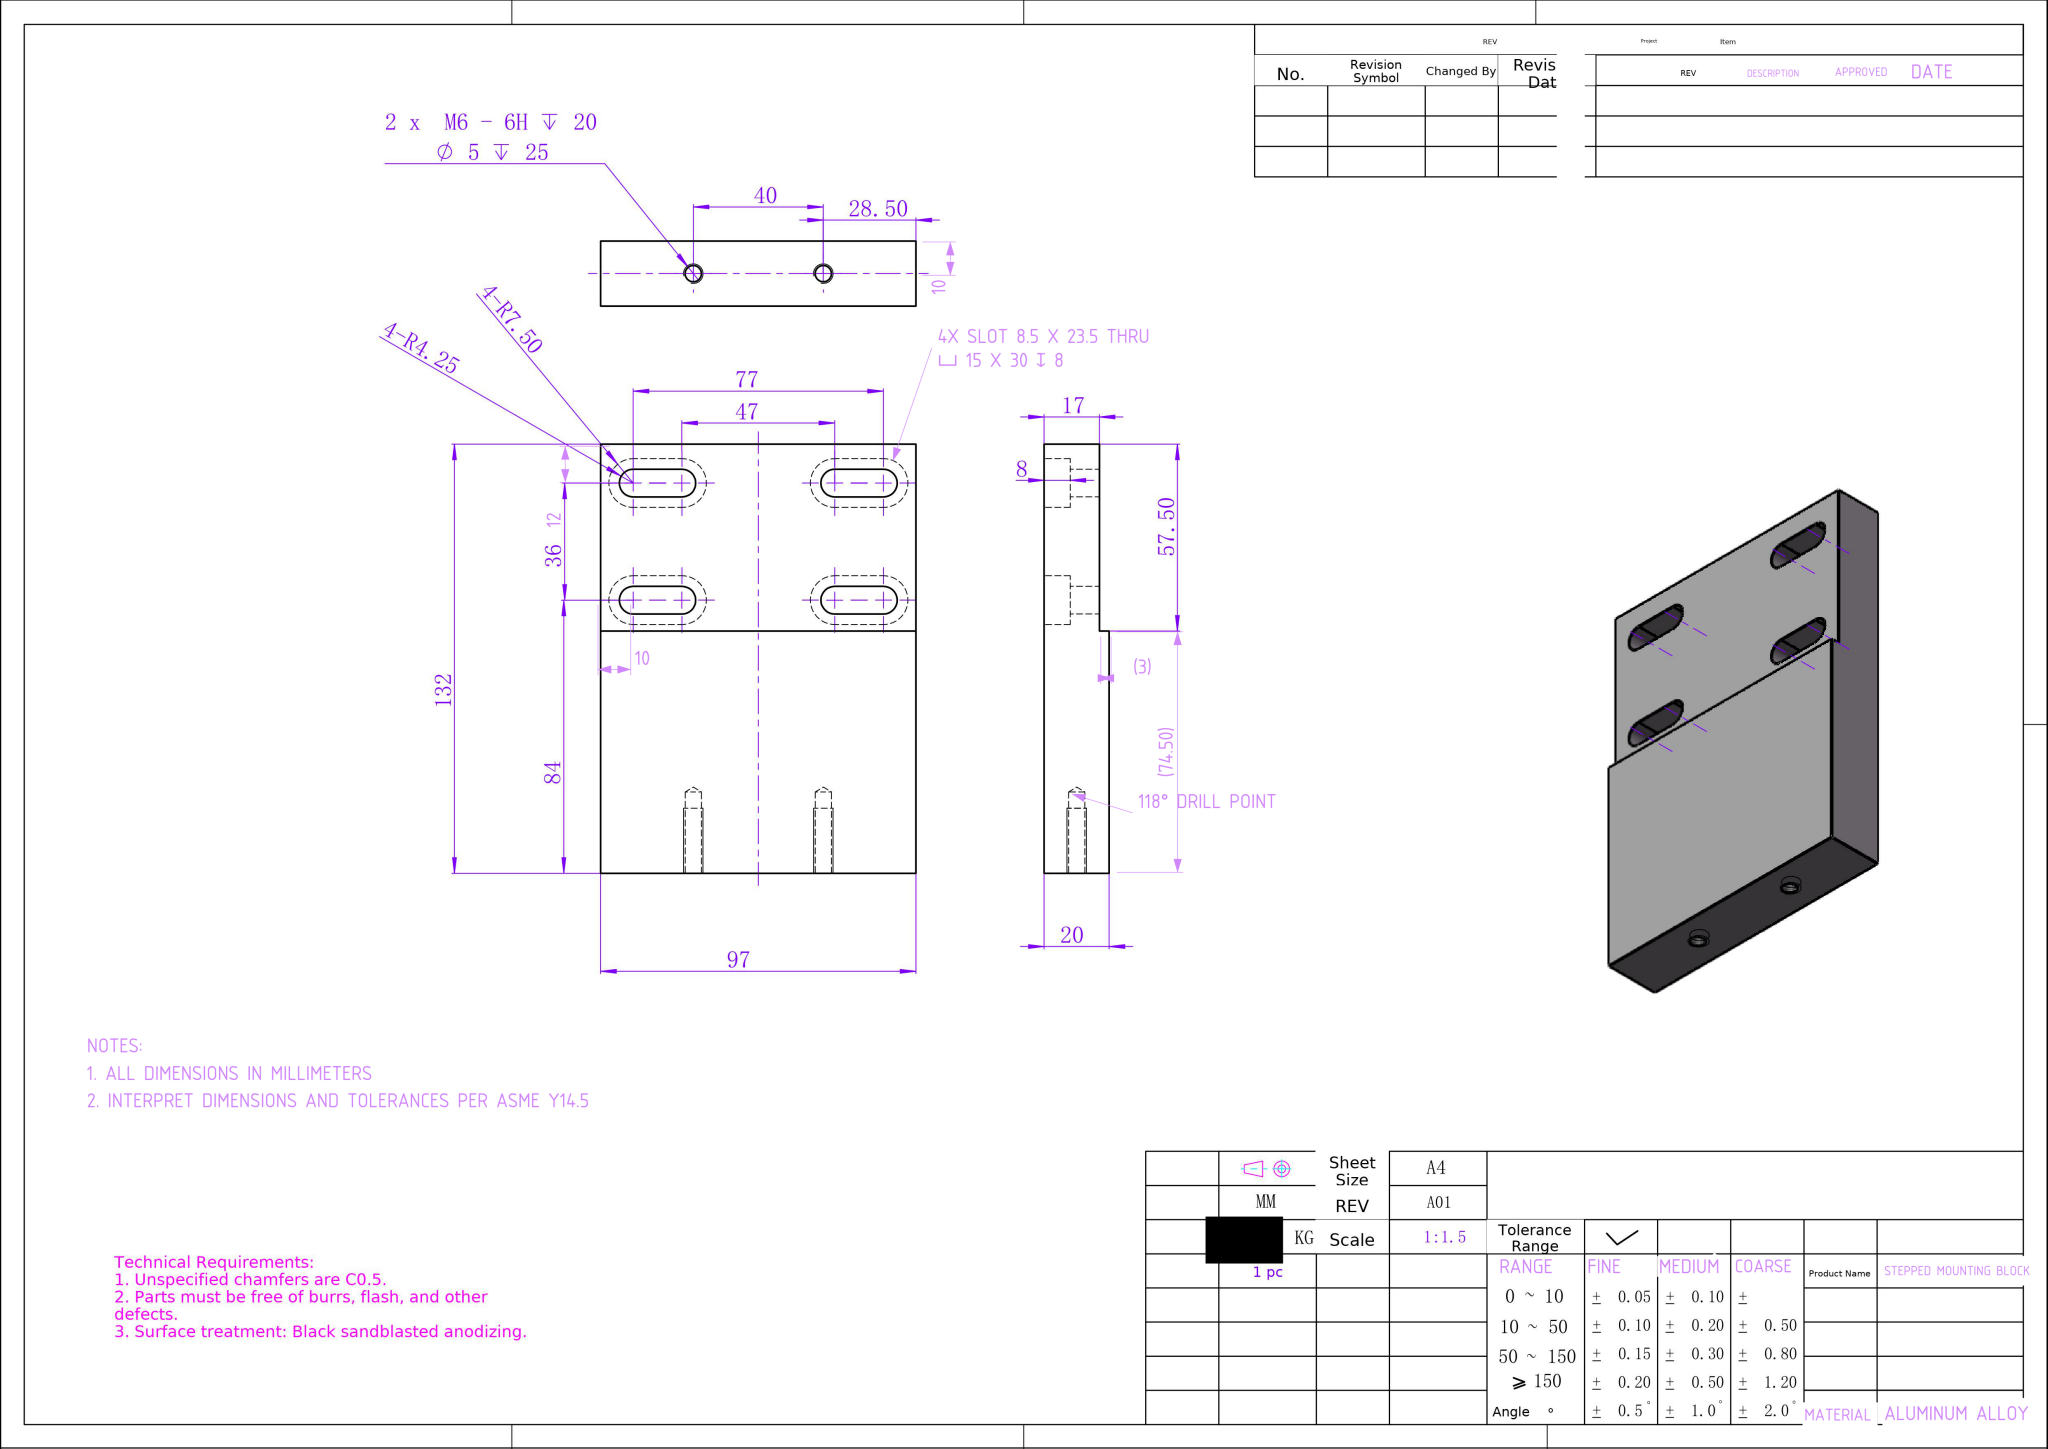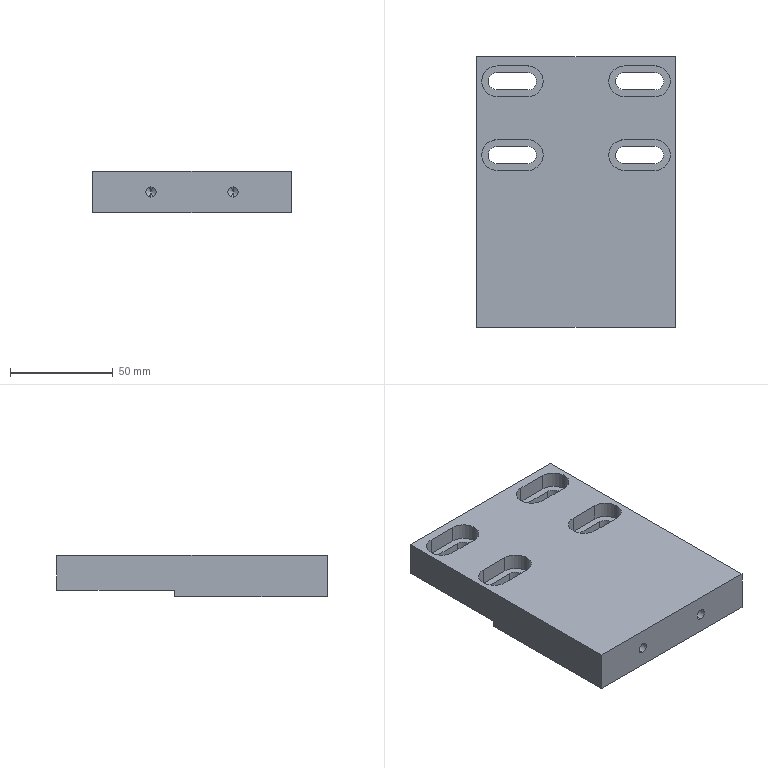Part | NX | mm | Quad-Slot Rectangular Base Plate | 1 solid | 60 faces | box 97 x 132 x 20 mm | volume 218858 mm3 | cylinder 28 | plane 28 | cone 4 | commonest cylinder face diameters 15 x12 8.5 x12 5 x4